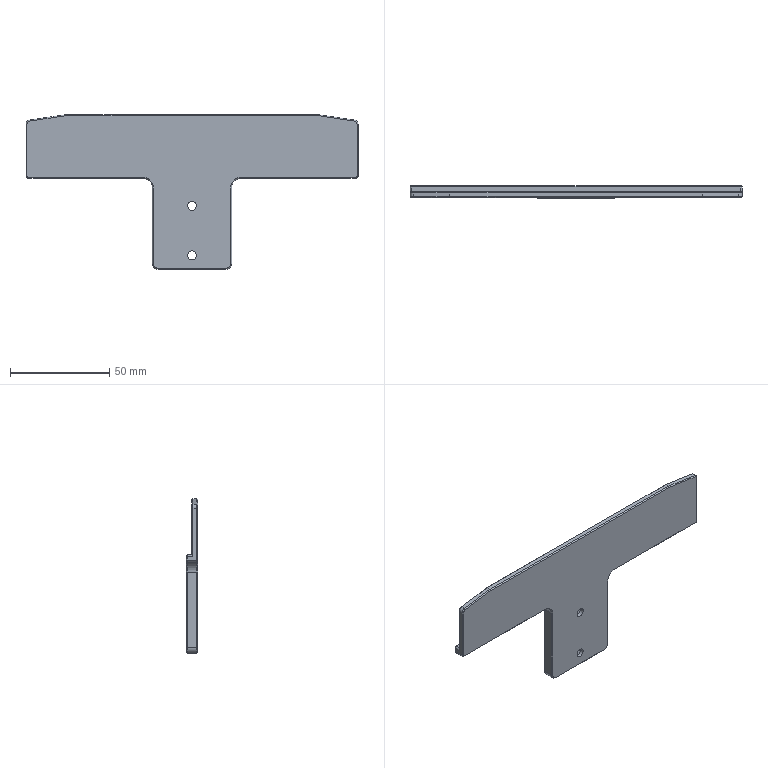Component | SolidWorks | SL010-LeftStreamline-1-1_SL010-SideClampAssembly-DB-1-1_SL010-LXFB-020200-020-1-1 | 1 solid | 78 faces | volume 28378 mm3 | plane 39 | cone 20 | cylinder 19 | commonest cylinder face diameters 8 x4 4.5 x4 2 x4 4 x3 10 x2 6 x2 | material Aluminum-6061